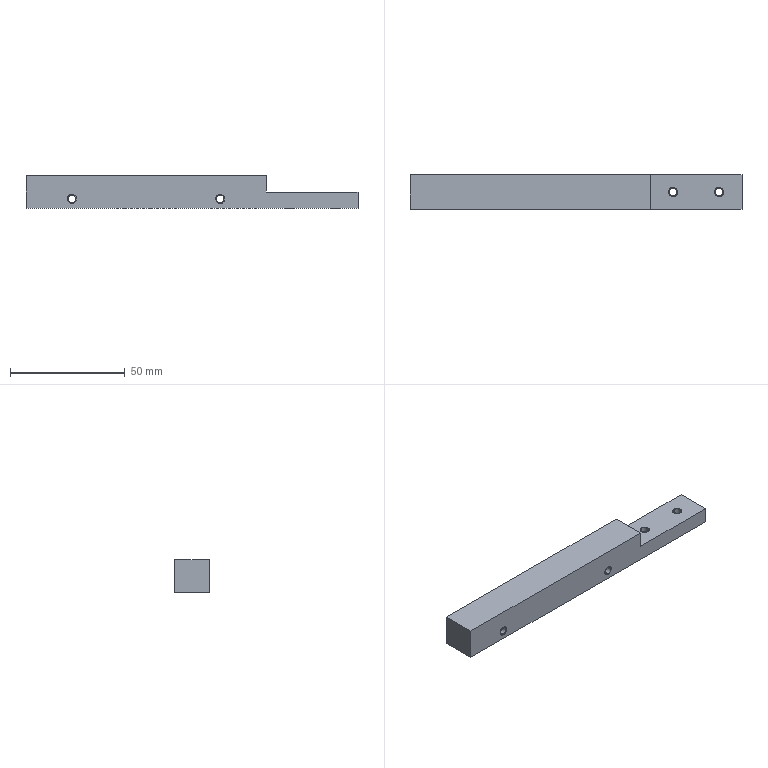CAM job | Mastercam | mm | 11 operations | part box 144.5 x 15 x 14
1. Facing | 24 - 50 平铣刀
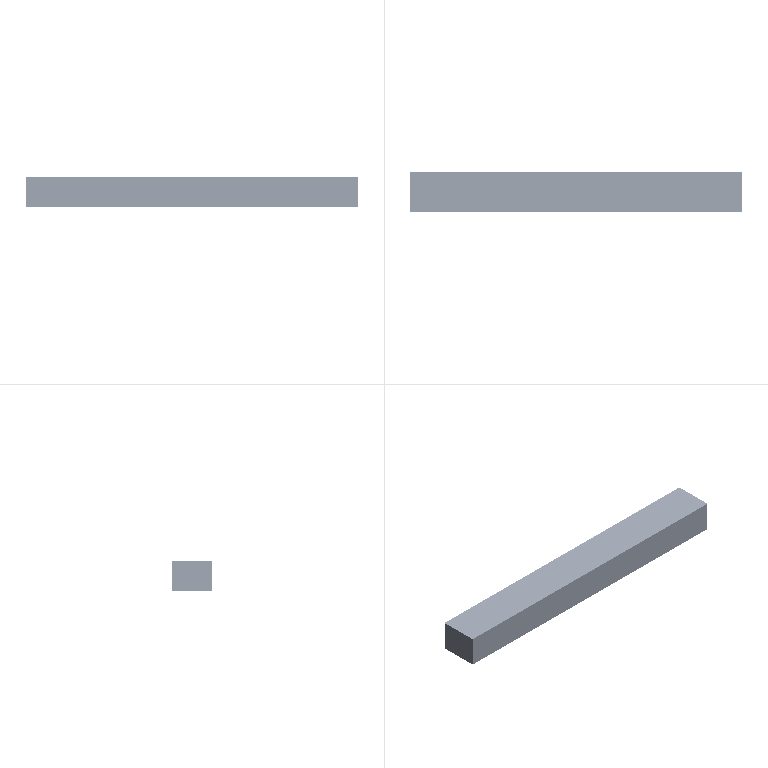2. Contour (Ramp) | 10 - 10 平铣刀
3. Contour (2D) | 10 - 10 平铣刀
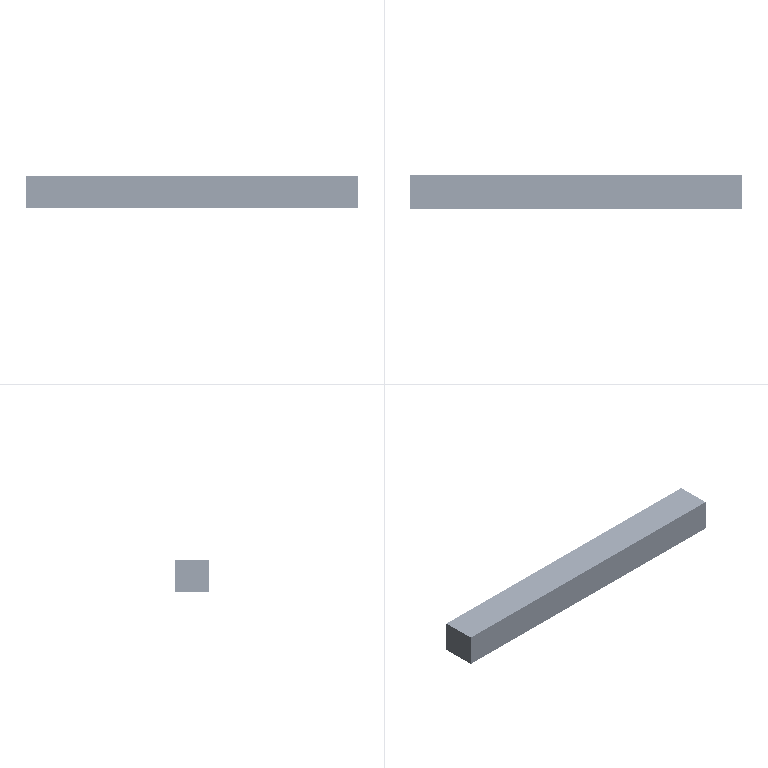4. Contour (2D chamfer) | 7 - 6 倒角刀
5. Facing | 24 - 50 平铣刀
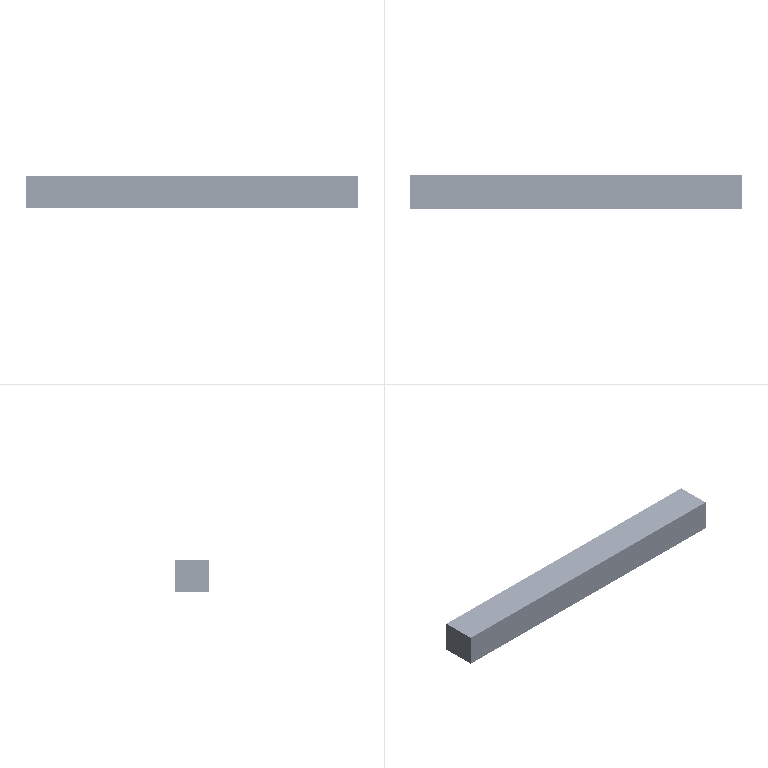6. Contour (Ramp) | 10 - 10 平铣刀
7. Contour (2D) | 10 - 10 平铣刀
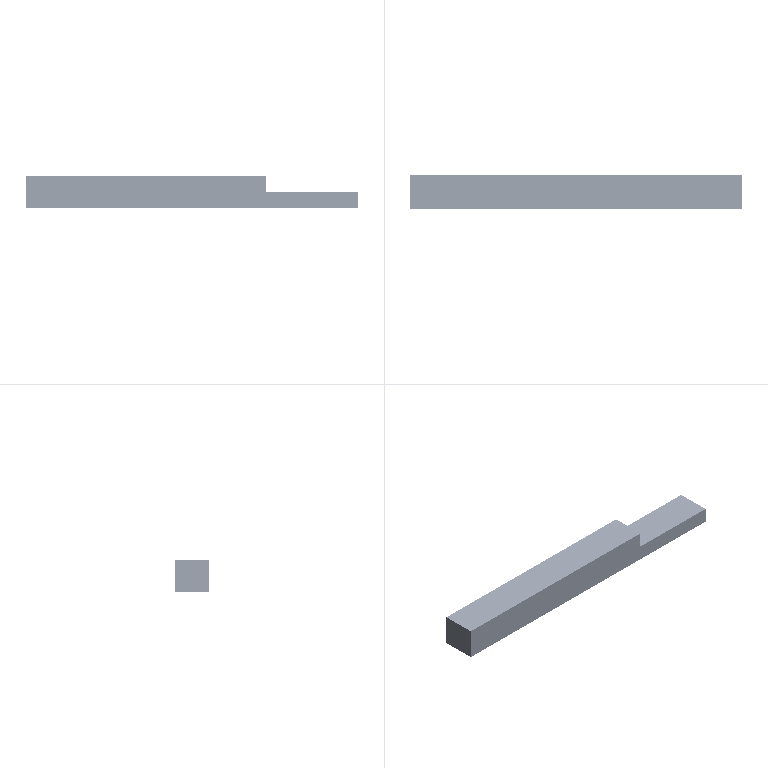8. Contour (2D chamfer) | 7 - 6 倒角刀
9. Contour (2D chamfer) | 7 - 6 倒角刀
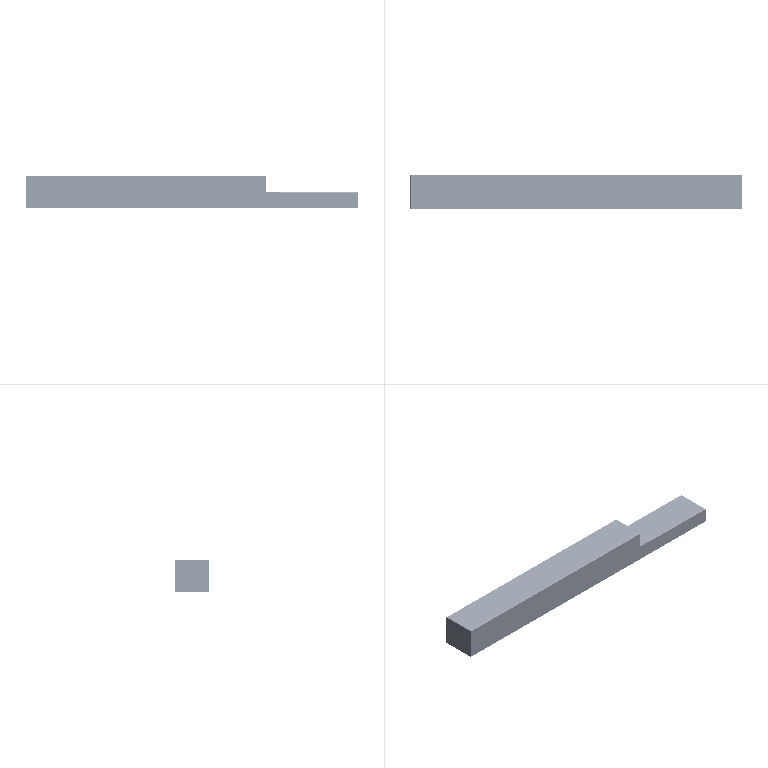10. Drill/Counterbore | 7 - 6 倒角刀
11. Drill/Counterbore | 7 - 6 倒角刀